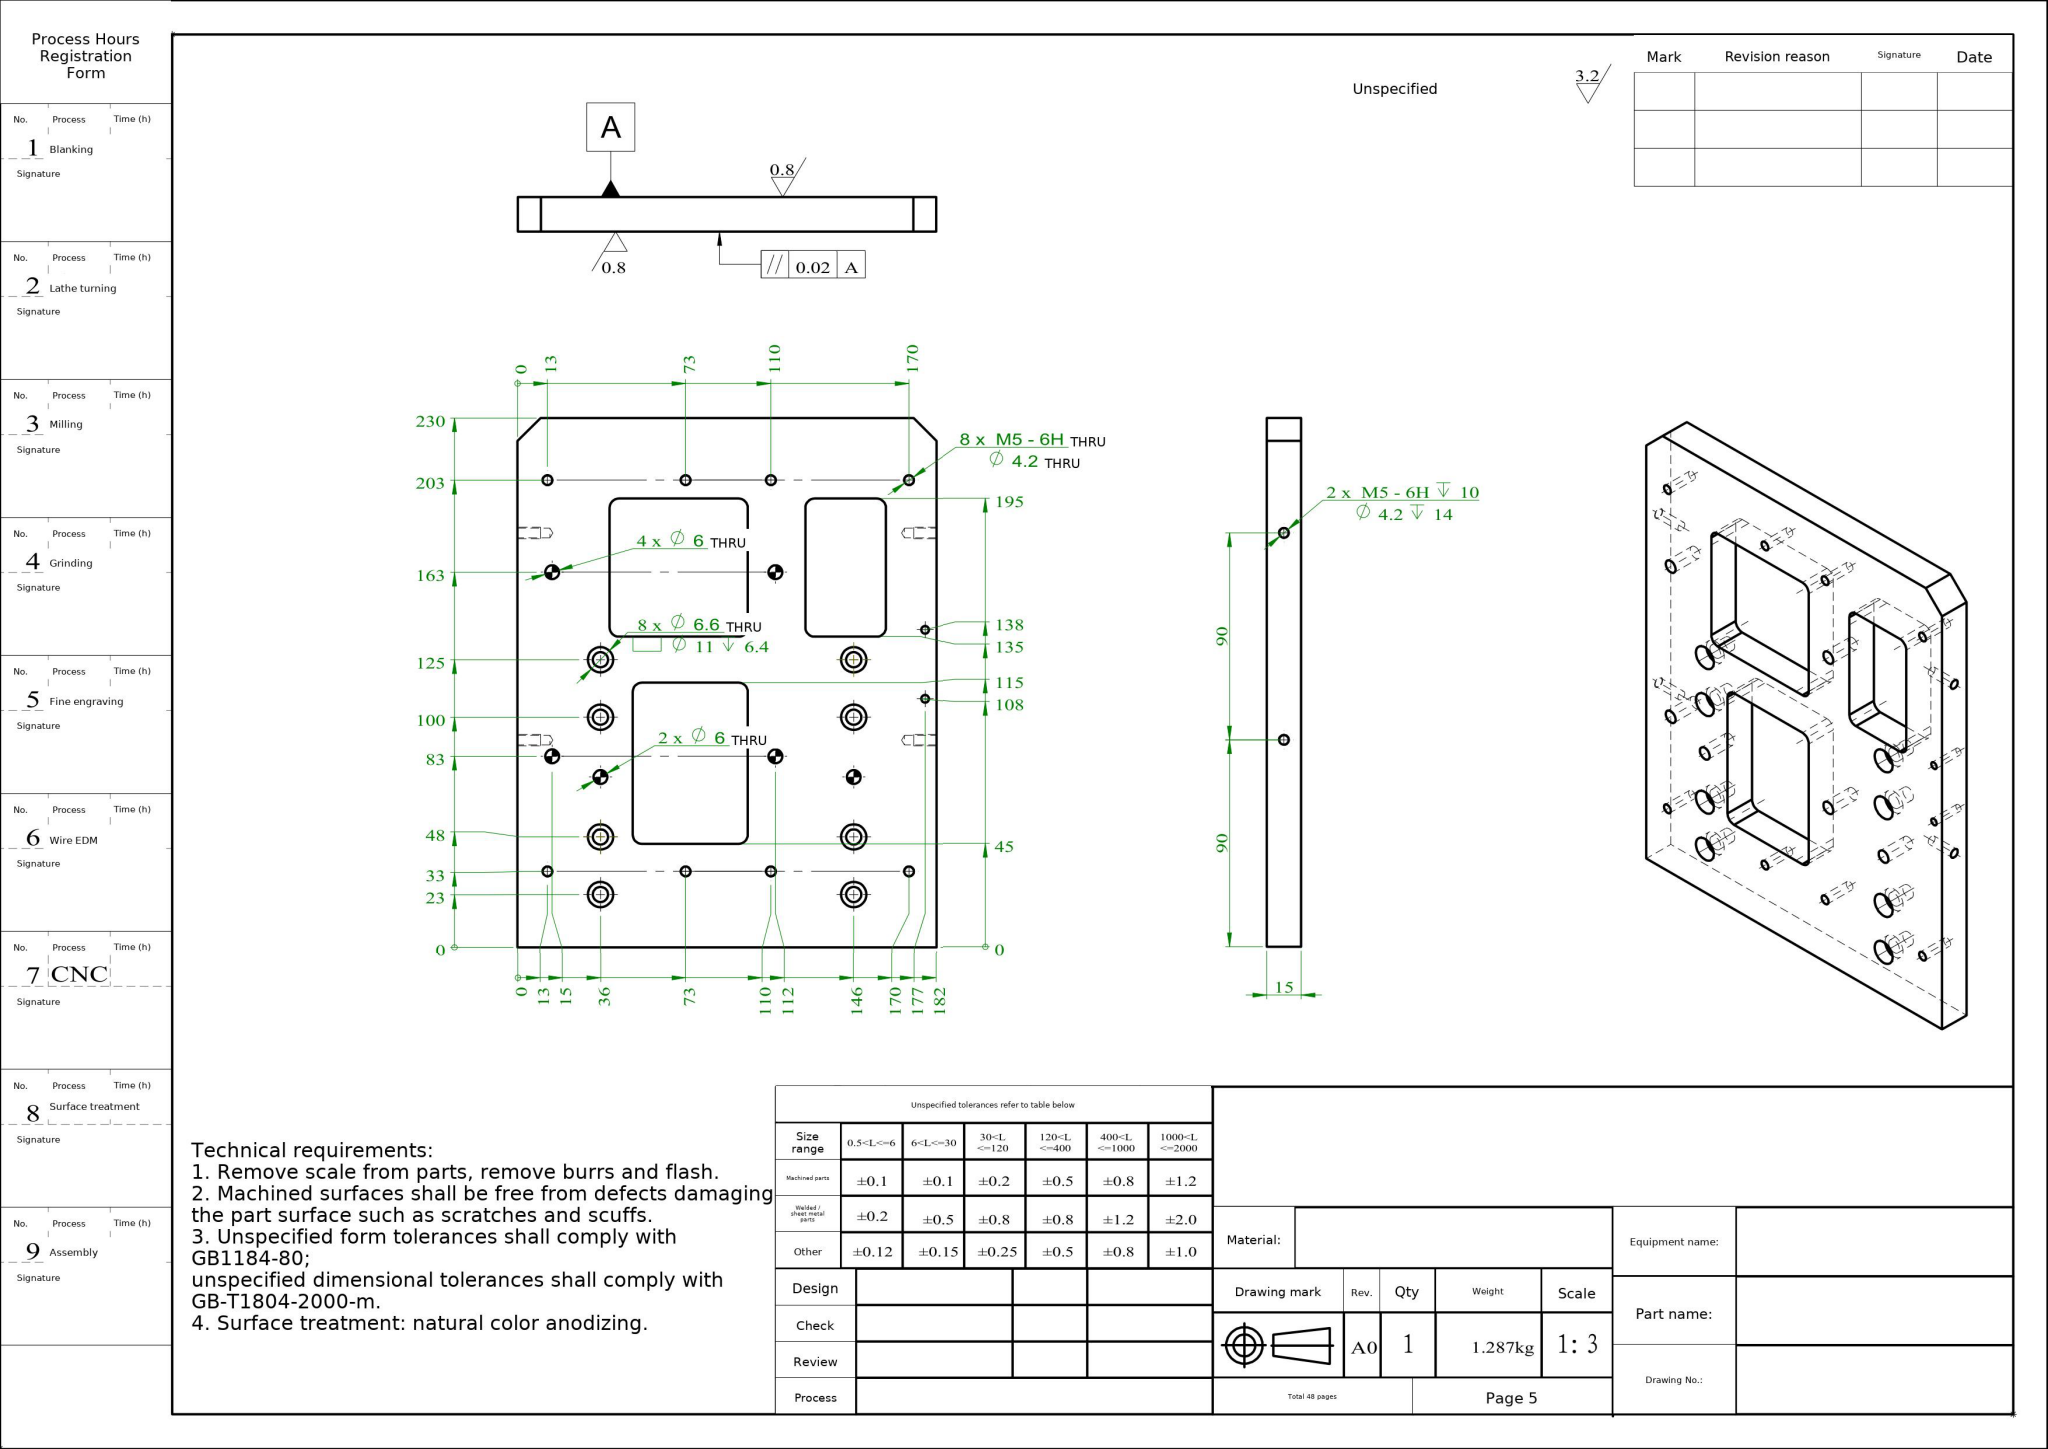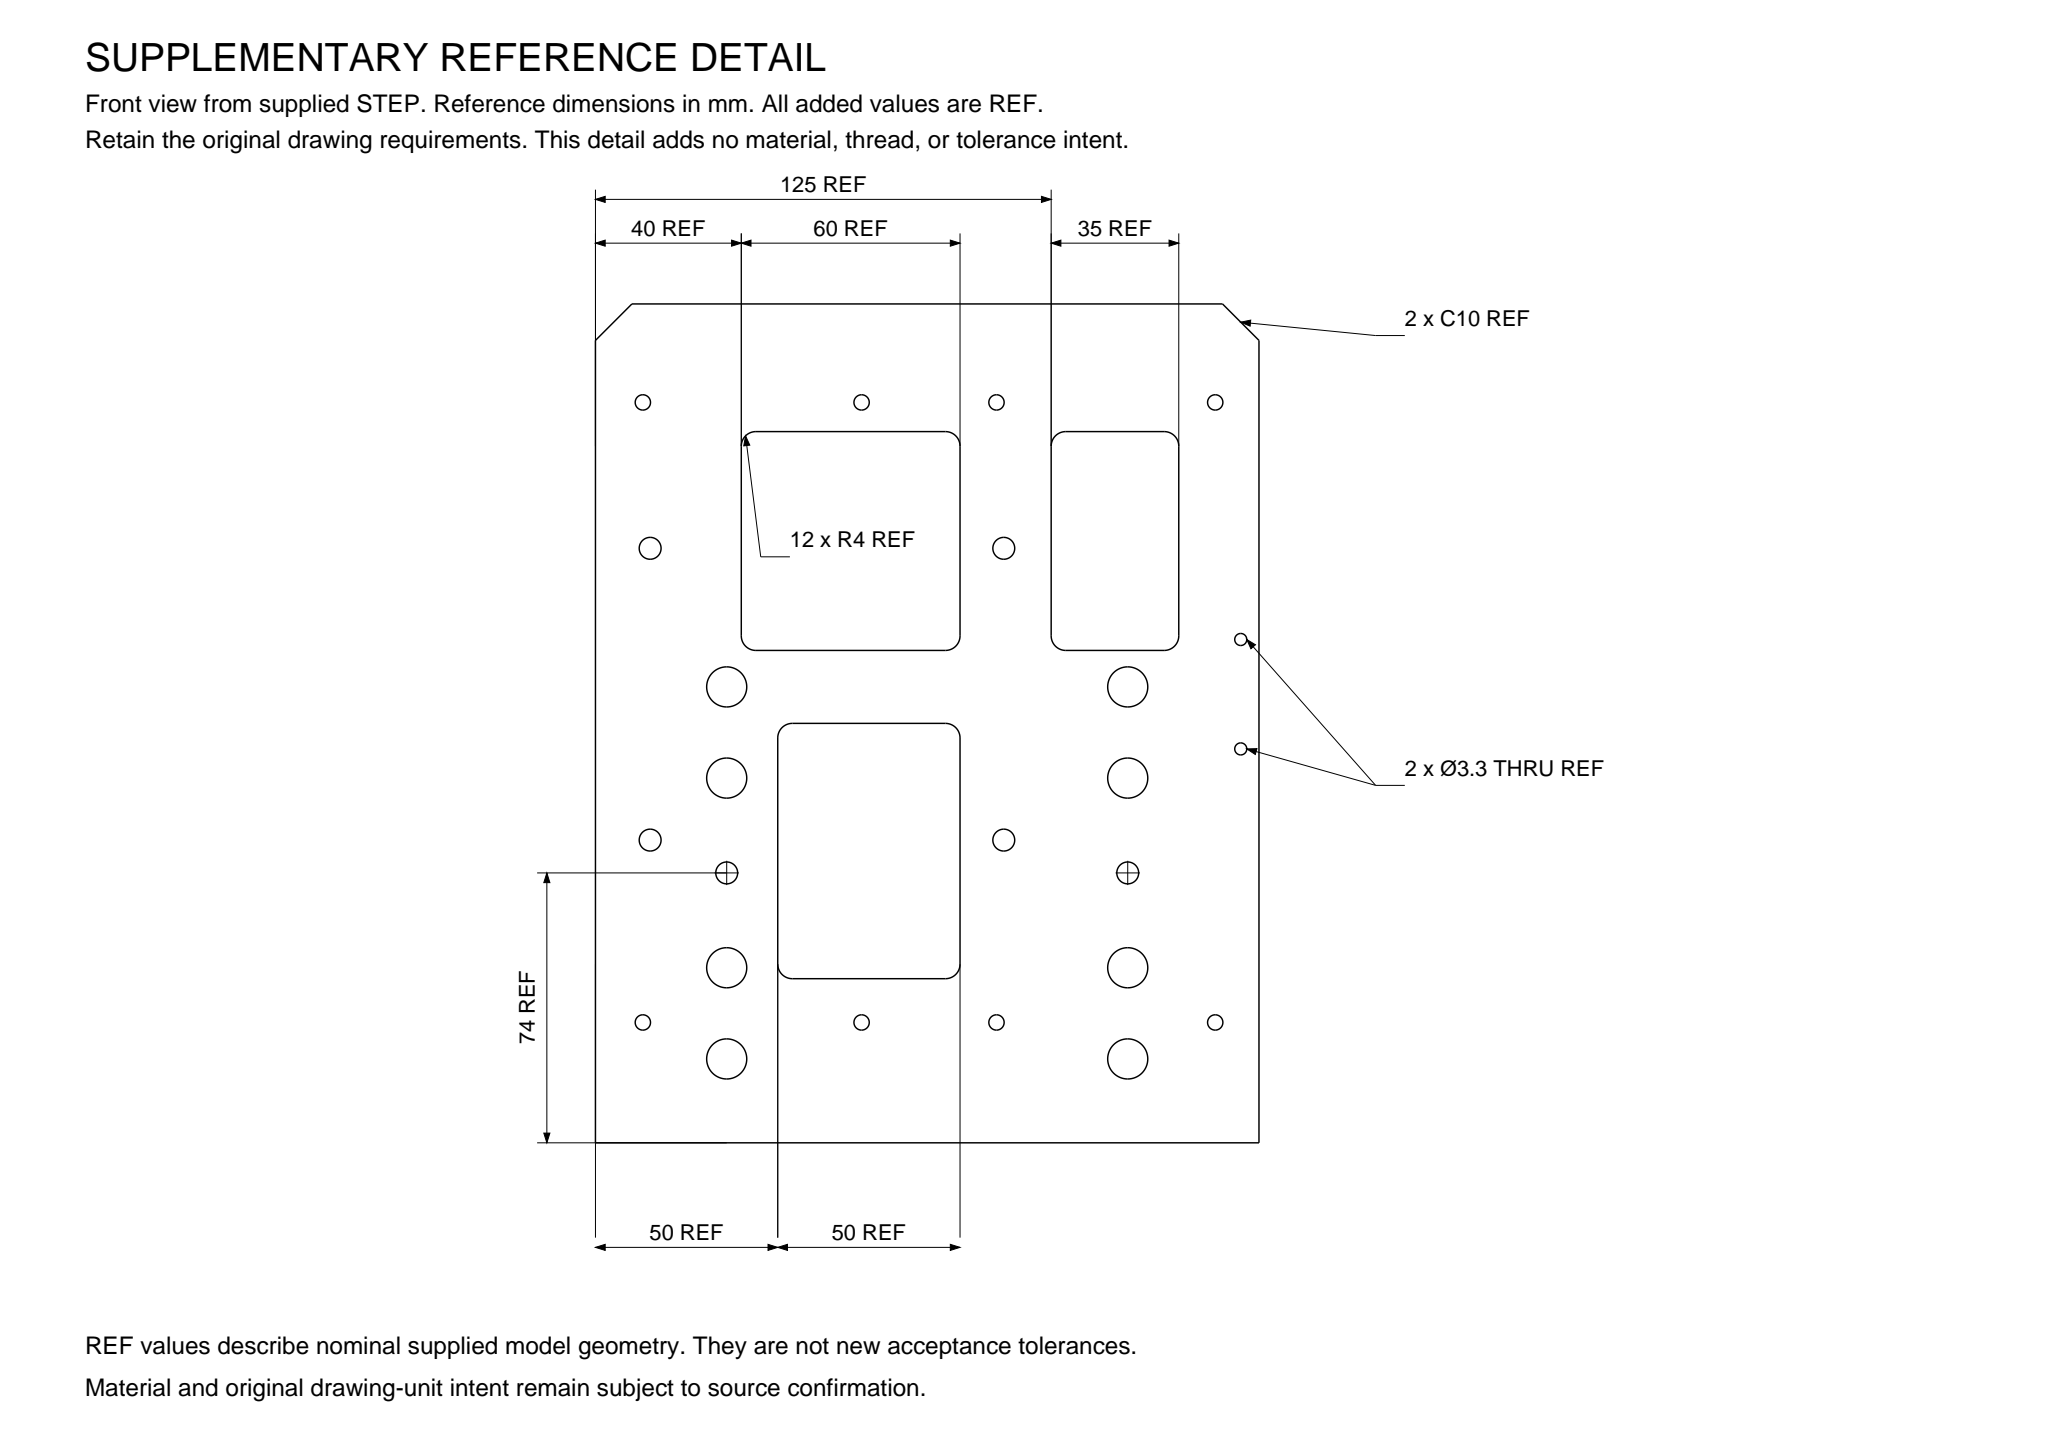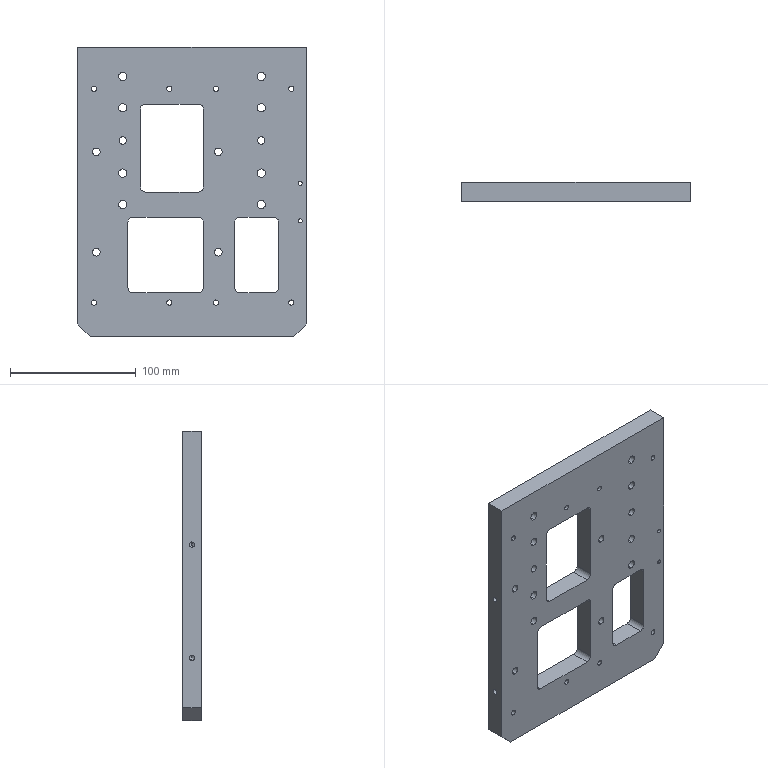Part | SolidWorks | mm | 1 solid | 120 faces | box 182 x 15 x 230 mm | volume 476536 mm3 | cylinder 84 | plane 28 | cone 8 | commonest cylinder face diameters 4.2 x24 11 x16 6.6 x16 6 x12 8 x12 3.3 x4